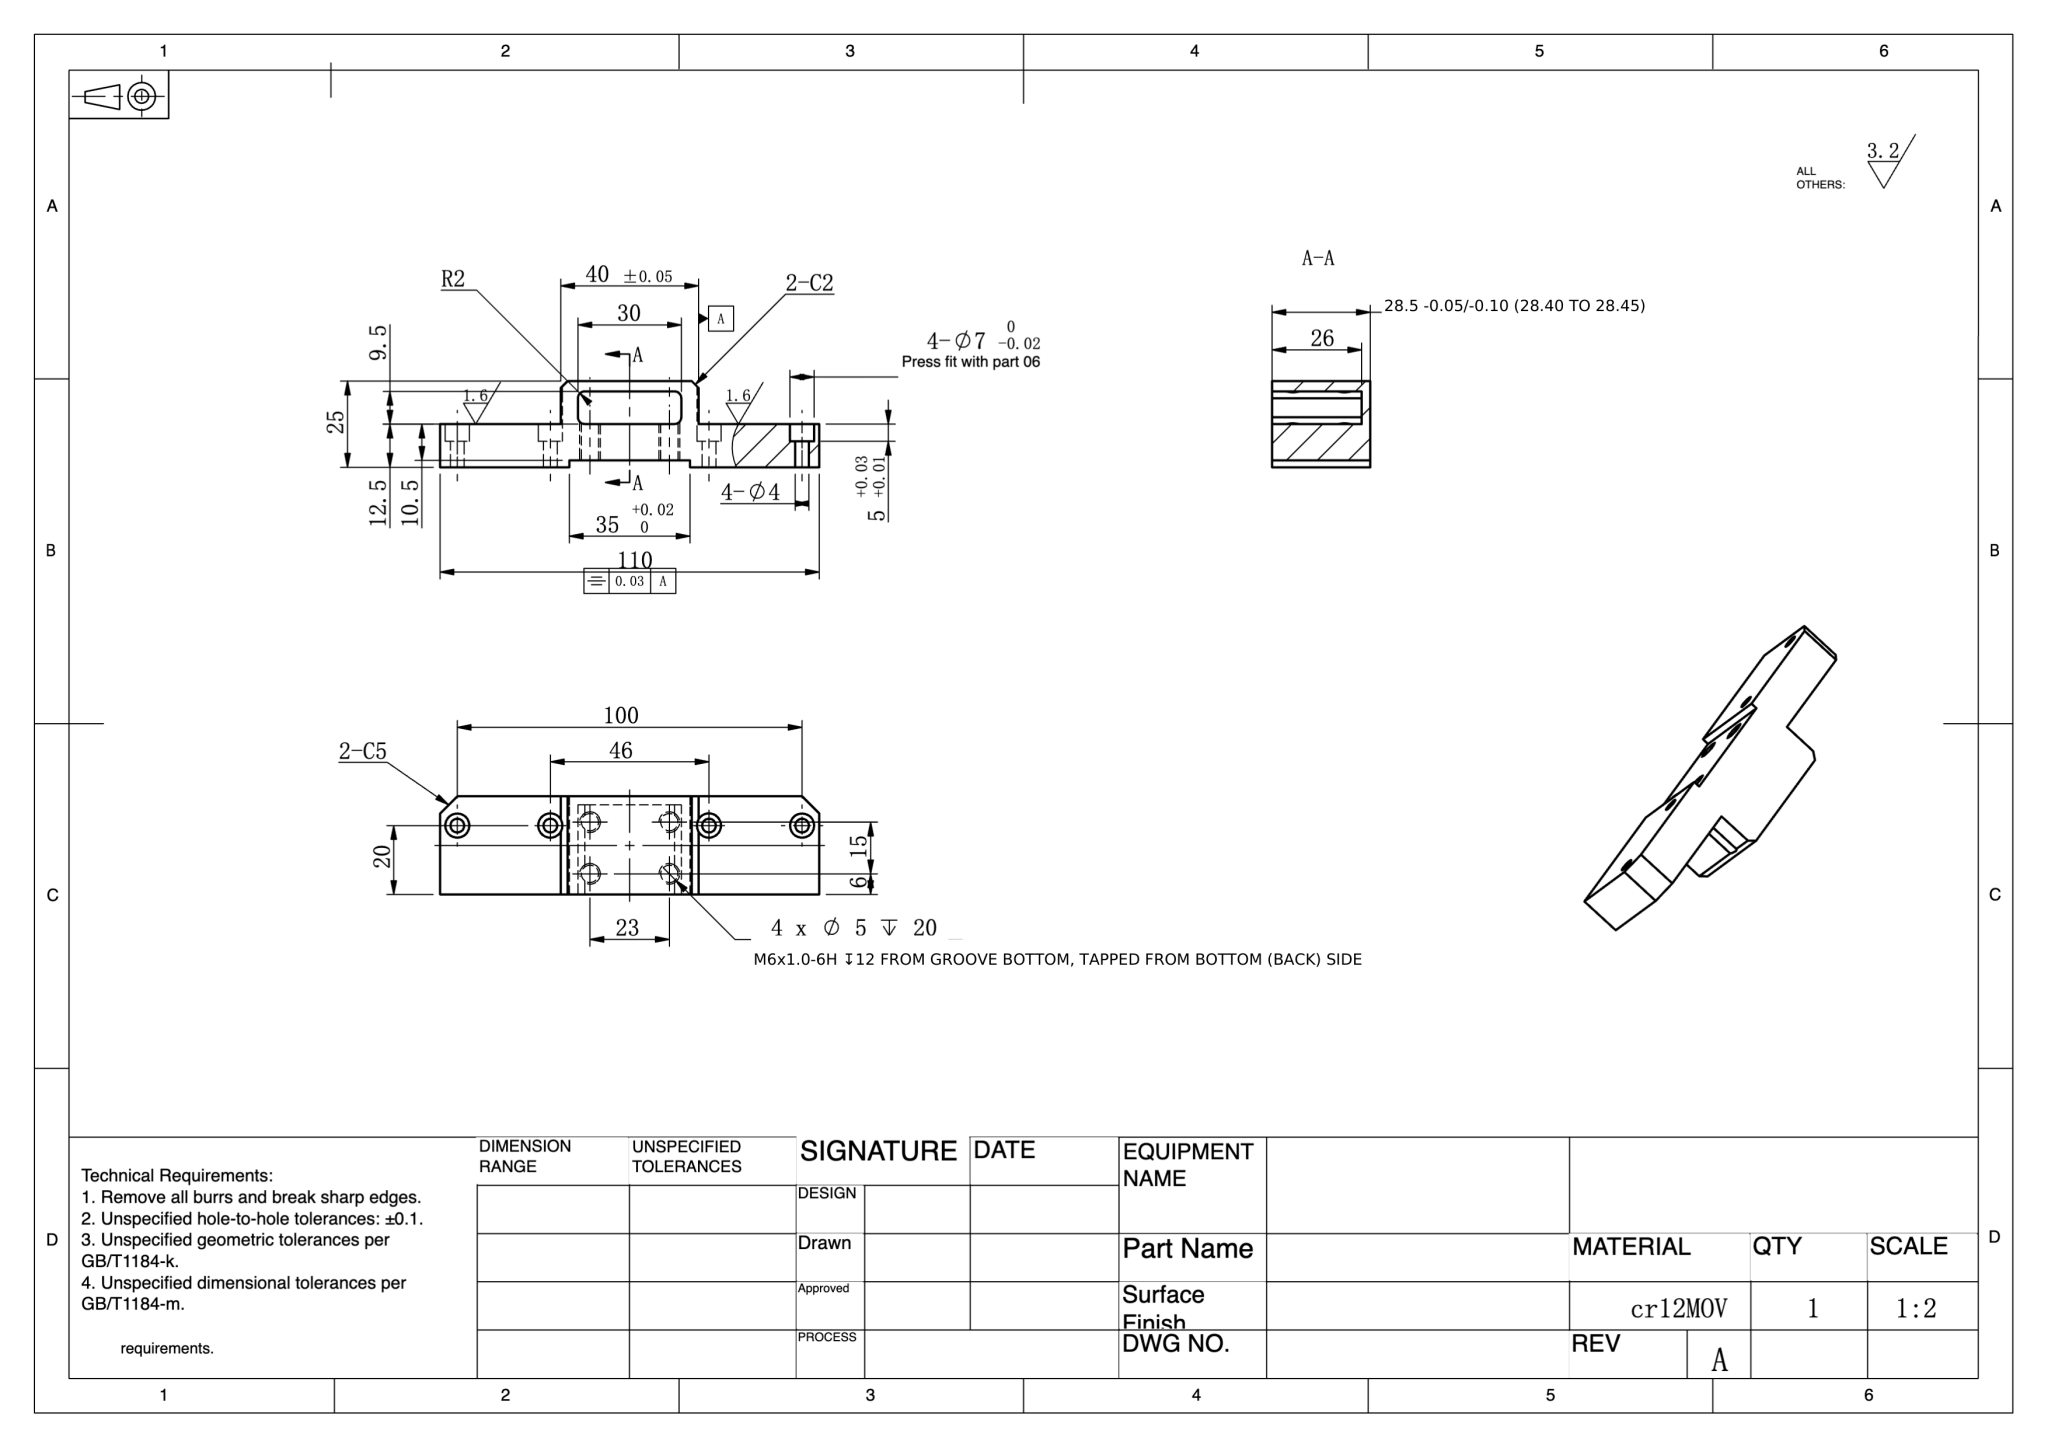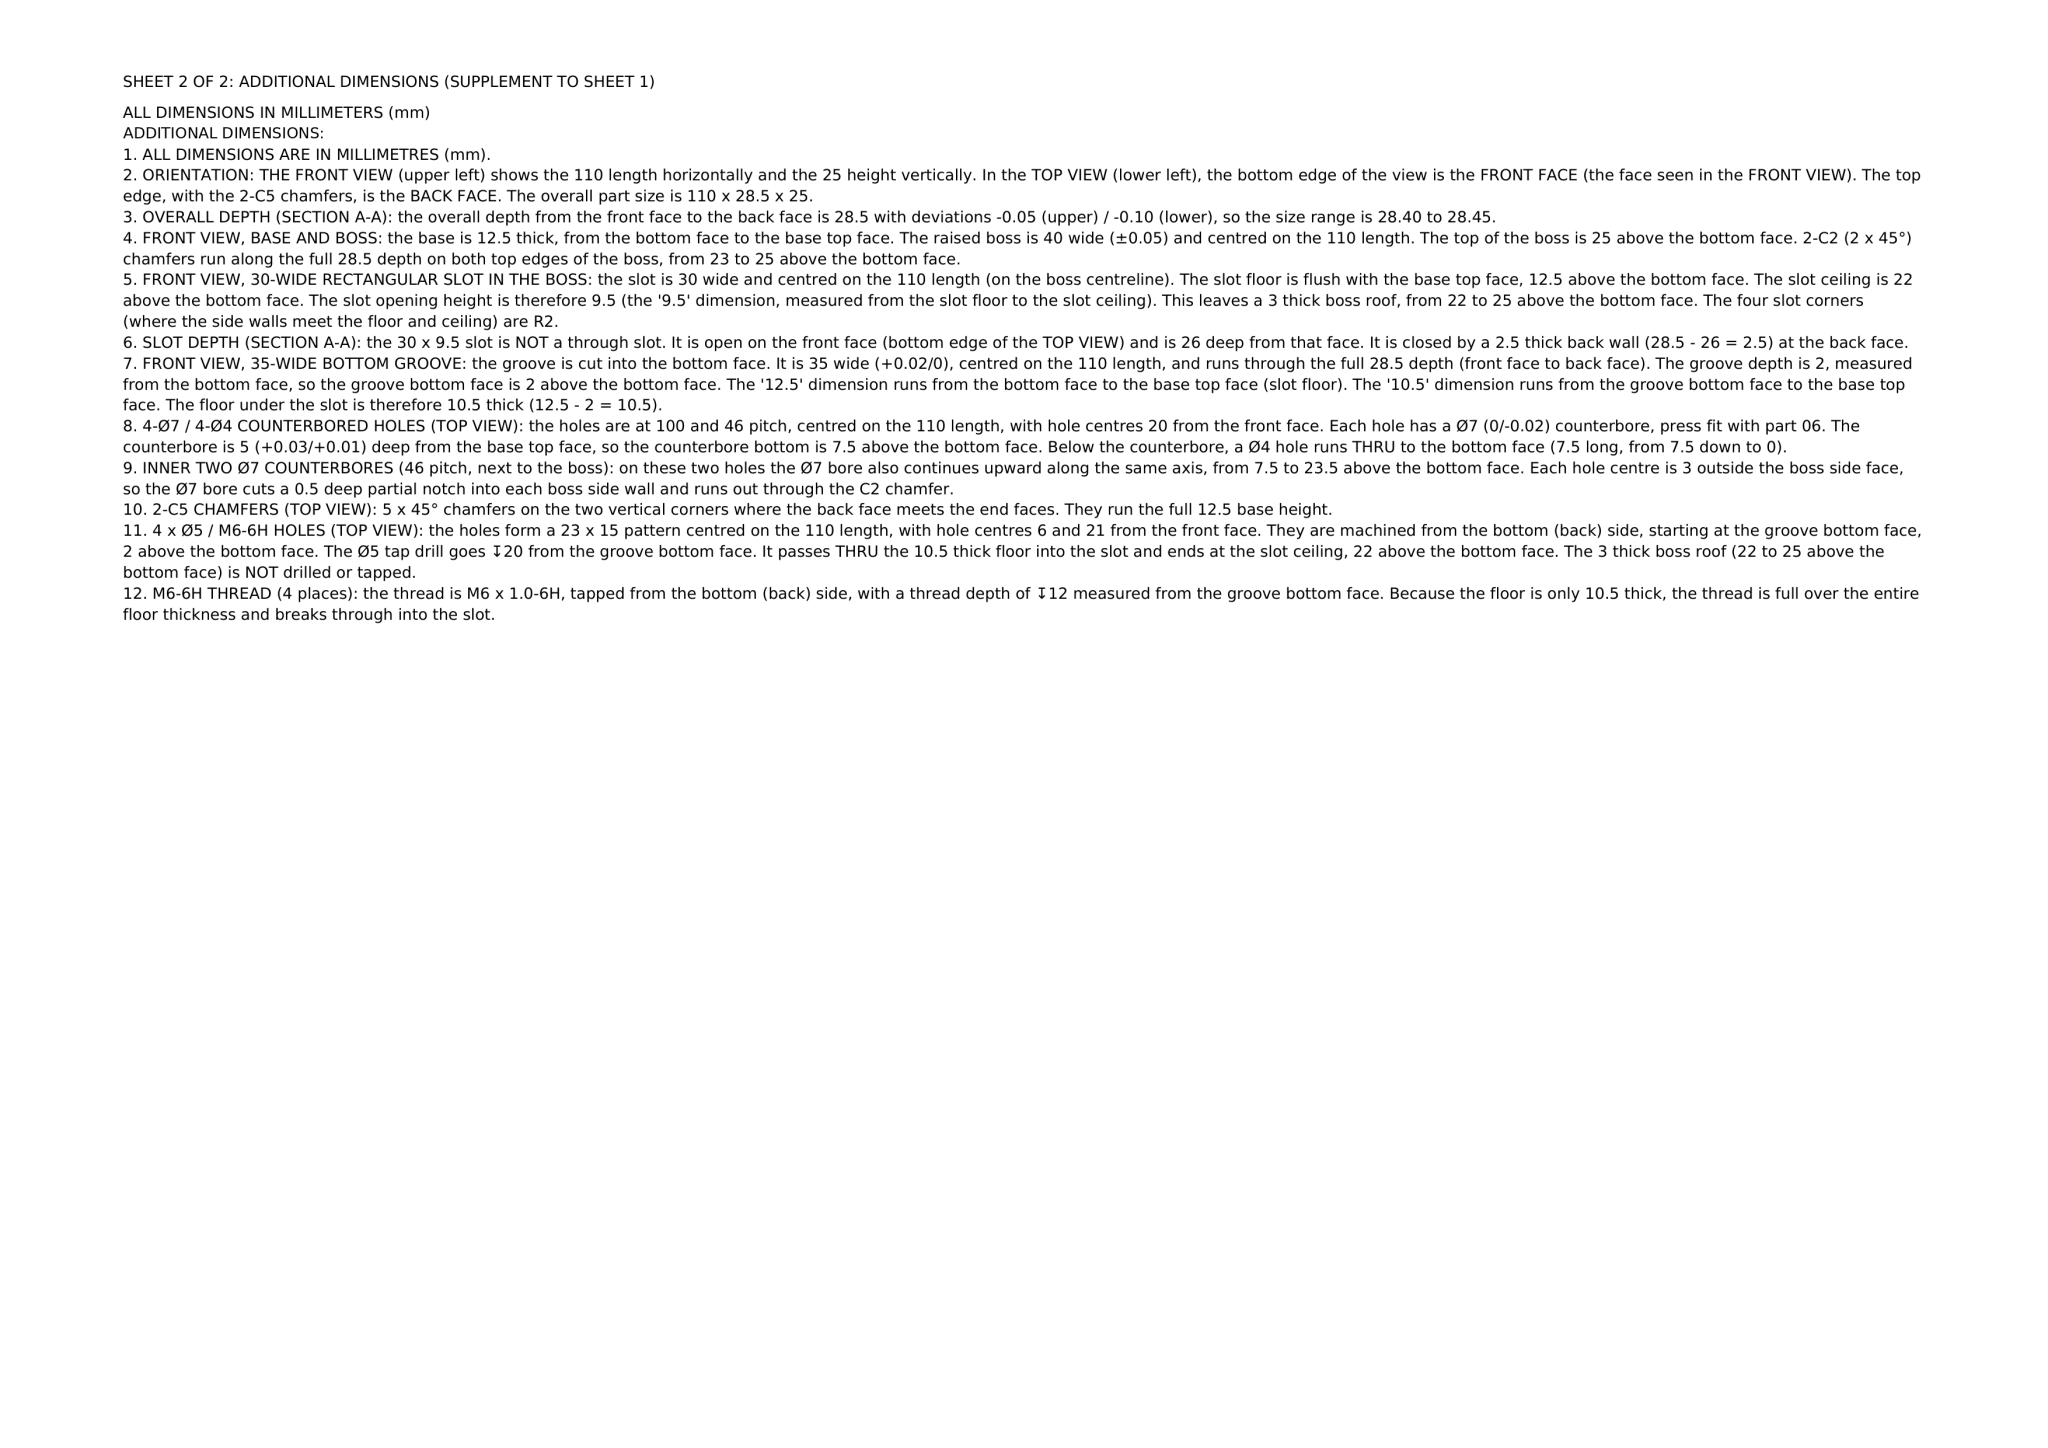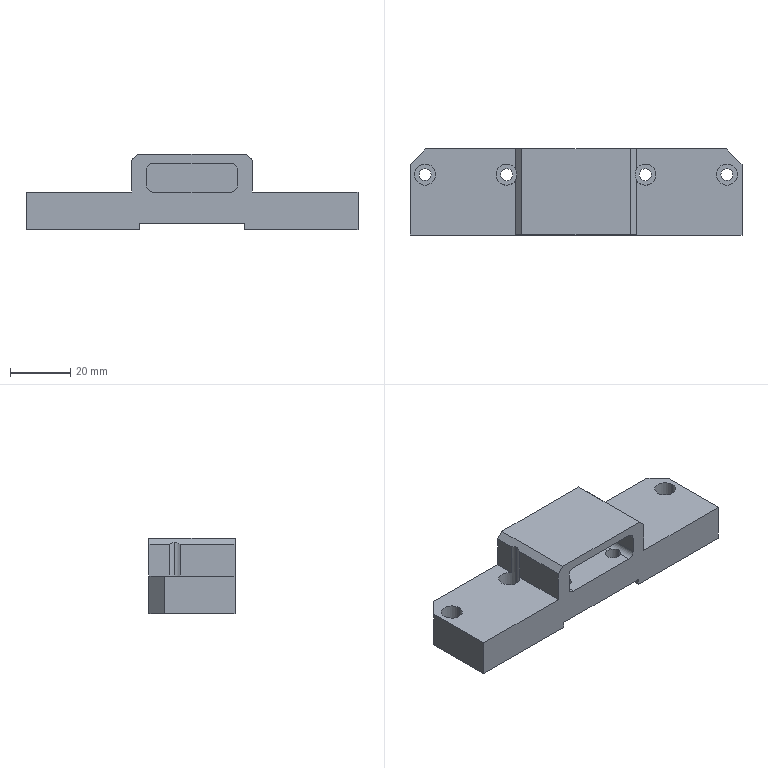Part | NX | mm | 1 solid | 63 faces | box 110 x 28.5 x 25 mm | volume 41696 mm3 | cylinder 34 | plane 29 | commonest cylinder face diameters 5 x14 4 x12 7 x8